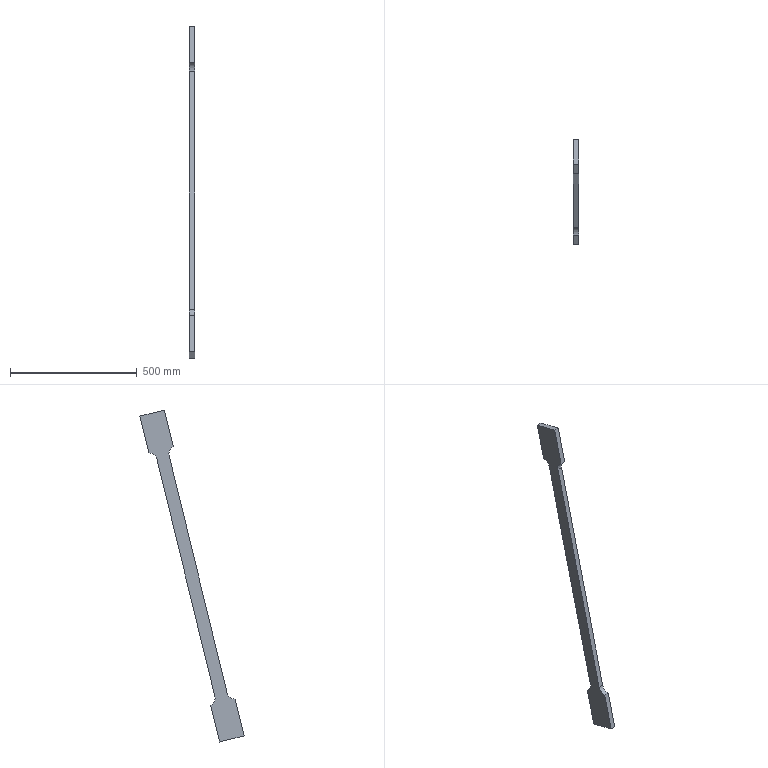Component | SolidWorks | Bocna spona oslonca izbacivaca-1 | 1 solid | 14 faces | box 20 x 412.18 x 1310.78 mm | volume 1639556 mm3 | plane 10 | cylinder 4 | commonest cylinder face diameters 60 x4
build123d program:
from build123d import *

# Parameters (mm, degrees)
BOSS_EXTRUDE1_DEPTH = 20


with BuildPart() as part:
    # Sketch1 → Boss-Extrude1 (new body)
    with BuildSketch(Plane(origin=(-5.82, 0, 0), x_dir=(0, 0, -1), z_dir=(1, 0, 0))):
        with BuildLine():
            Line((-662.5, 50), (-662.5, -50))
            Line((-662.5, -50), (-512.5, -50))
            ThreePointArc((-512.5, -50), (-502.285, -32.087), (-482.92, -25))
            Line((-482.92, -25), (482.92, -25))
            ThreePointArc((482.92, -25), (502.285, -32.087), (512.5, -50))
            Line((512.5, -50), (662.5, -50))
            Line((662.5, -50), (662.5, 50))
            Line((662.5, 50), (512.5, 50))
            ThreePointArc((512.5, 50), (502.285, 32.087), (482.92, 25))
            Line((482.92, 25), (-482.92, 25))
            ThreePointArc((-482.92, 25), (-502.285, 32.087), (-512.5, 50))
            Line((-512.5, 50), (-662.5, 50))
        make_face()
    extrude(amount=BOSS_EXTRUDE1_DEPTH)


solid = part.part

# Placed as in the assembly
solid = solid.moved(Location((6.82, 160.049, -734.493), (166.245, 0, 0)))
STEP:
#1=COLOUR_RGB('',0.7922,0.8196,0.9333);
#2=FILL_AREA_STYLE_COLOUR('',#1);
#3=FILL_AREA_STYLE('',(#2));
#4=SURFACE_STYLE_FILL_AREA(#3);
#5=SURFACE_SIDE_STYLE('',(#4));
#6=SURFACE_STYLE_USAGE(.BOTH.,#5);
#7=PRESENTATION_STYLE_ASSIGNMENT((#6));
#8=CARTESIAN_POINT('',(0.03937,3.416,-48.984));
#9=VERTEX_POINT('',#8);
#10=CARTESIAN_POINT('',(0.03937,2.737,-47.618));
#11=VERTEX_POINT('',#10);
#12=CARTESIAN_POINT('',(0.03937,3.884,-47.899));
#13=DIRECTION('',(-1.,-0.,-0.));
#14=DIRECTION('',(0.,-0.2378,-0.9713));
#15=AXIS2_PLACEMENT_3D('',#12,#13,#14);
#16=CIRCLE('',#15,1.181);
#17=EDGE_CURVE('',#9,#11,#16,.T.);
#18=ORIENTED_EDGE('',*,*,#17,.T.);
#19=CARTESIAN_POINT('',(0.8268,2.737,-47.618));
#20=VERTEX_POINT('',#19);
#21=CARTESIAN_POINT('',(0.8268,2.737,-47.618));
#22=DIRECTION('',(-1.,-0.,-0.));
#23=VECTOR('',#22,39.37);
#24=LINE('',#21,#23);
#25=EDGE_CURVE('',#20,#11,#24,.T.);
#26=ORIENTED_EDGE('',*,*,#25,.F.);
#27=CARTESIAN_POINT('',(0.8268,3.416,-48.984));
#28=VERTEX_POINT('',#27);
#29=CARTESIAN_POINT('',(0.8268,3.884,-47.899));
#30=DIRECTION('',(-1.,-0.,-0.));
#31=DIRECTION('',(0.,-0.2378,-0.9713));
#32=AXIS2_PLACEMENT_3D('',#29,#30,#31);
#33=CIRCLE('',#32,1.181);
#34=EDGE_CURVE('',#28,#20,#33,.T.);
#35=ORIENTED_EDGE('',*,*,#34,.F.);
#36=CARTESIAN_POINT('',(0.8268,3.416,-48.984));
#37=DIRECTION('',(-1.,-0.,-0.));
#38=VECTOR('',#37,39.37);
#39=LINE('',#36,#38);
#40=EDGE_CURVE('',#28,#9,#39,.T.);
#41=ORIENTED_EDGE('',*,*,#40,.T.);
#42=EDGE_LOOP('',(#18,#26,#35,#41));
#43=FACE_OUTER_BOUND('',#42,.T.);
#44=CARTESIAN_POINT('',(0.8268,3.884,-47.899));
#45=DIRECTION('',(-1.,-0.,-0.));
#46=DIRECTION('',(0.,0.2378,0.9713));
#47=AXIS2_PLACEMENT_3D('',#44,#45,#46);
#48=CYLINDRICAL_SURFACE('',#47,1.181);
#49=ADVANCED_FACE('',(#43),#48,.F.);
#50=CARTESIAN_POINT('',(0.03937,11.778,-10.684));
#51=VERTEX_POINT('',#50);
#52=CARTESIAN_POINT('',(0.03937,11.778,-10.684));
#53=DIRECTION('',(-0.,0.2378,0.9713));
#54=VECTOR('',#53,39.37);
#55=LINE('',#52,#54);
#56=EDGE_CURVE('',#11,#51,#55,.T.);
#57=ORIENTED_EDGE('',*,*,#56,.T.);
#58=CARTESIAN_POINT('',(0.8268,11.778,-10.684));
#59=VERTEX_POINT('',#58);
#60=CARTESIAN_POINT('',(0.8268,11.778,-10.684));
#61=DIRECTION('',(-1.,-0.,-0.));
#62=VECTOR('',#61,39.37);
#63=LINE('',#60,#62);
#64=EDGE_CURVE('',#59,#51,#63,.T.);
#65=ORIENTED_EDGE('',*,*,#64,.F.);
#66=CARTESIAN_POINT('',(0.8268,11.778,-10.684));
#67=DIRECTION('',(-0.,0.2378,0.9713));
#68=VECTOR('',#67,39.37);
#69=LINE('',#66,#68);
#70=EDGE_CURVE('',#20,#59,#69,.T.);
#71=ORIENTED_EDGE('',*,*,#70,.F.);
#72=ORIENTED_EDGE('',*,*,#25,.T.);
#73=EDGE_LOOP('',(#57,#65,#71,#72));
#74=FACE_OUTER_BOUND('',#73,.T.);
#75=CARTESIAN_POINT('',(0.8268,11.778,-10.684));
#76=DIRECTION('',(-0.,-0.9713,0.2378));
#77=DIRECTION('',(1.,-0.,0.));
#78=AXIS2_PLACEMENT_3D('',#75,#76,#77);
#79=PLANE('',#78);
#80=ADVANCED_FACE('',(#74),#79,.F.);
#81=CARTESIAN_POINT('',(0.03937,13.011,-9.787));
#82=VERTEX_POINT('',#81);
#83=CARTESIAN_POINT('',(0.03937,12.925,-10.965));
#84=DIRECTION('',(-1.,-0.,-0.));
#85=DIRECTION('',(-0.,0.2378,0.9713));
#86=AXIS2_PLACEMENT_3D('',#83,#84,#85);
#87=CIRCLE('',#86,1.181);
#88=EDGE_CURVE('',#51,#82,#87,.T.);
#89=ORIENTED_EDGE('',*,*,#88,.T.);
#90=CARTESIAN_POINT('',(0.8268,13.011,-9.787));
#91=VERTEX_POINT('',#90);
#92=CARTESIAN_POINT('',(0.8268,13.011,-9.787));
#93=DIRECTION('',(-1.,-0.,-0.));
#94=VECTOR('',#93,39.37);
#95=LINE('',#92,#94);
#96=EDGE_CURVE('',#91,#82,#95,.T.);
#97=ORIENTED_EDGE('',*,*,#96,.F.);
#98=CARTESIAN_POINT('',(0.8268,12.925,-10.965));
#99=DIRECTION('',(-1.,-0.,-0.));
#100=DIRECTION('',(0.,0.2378,0.9713));
#101=AXIS2_PLACEMENT_3D('',#98,#99,#100);
#102=CIRCLE('',#101,1.181);
#103=EDGE_CURVE('',#59,#91,#102,.T.);
#104=ORIENTED_EDGE('',*,*,#103,.F.);
#105=ORIENTED_EDGE('',*,*,#64,.T.);
#106=EDGE_LOOP('',(#89,#97,#104,#105));
#107=FACE_OUTER_BOUND('',#106,.T.);
#108=CARTESIAN_POINT('',(0.8268,12.925,-10.965));
#109=DIRECTION('',(-1.,-0.,-0.));
#110=DIRECTION('',(0.,0.2378,0.9713));
#111=AXIS2_PLACEMENT_3D('',#108,#109,#110);
#112=CYLINDRICAL_SURFACE('',#111,1.181);
#113=ADVANCED_FACE('',(#107),#112,.F.);
#114=CARTESIAN_POINT('',(0.03937,14.415,-4.05));
#115=VERTEX_POINT('',#114);
#116=CARTESIAN_POINT('',(0.03937,13.011,-9.787));
#117=DIRECTION('',(-0.,0.2378,0.9713));
#118=VECTOR('',#117,39.37);
#119=LINE('',#116,#118);
#120=EDGE_CURVE('',#82,#115,#119,.T.);
#121=ORIENTED_EDGE('',*,*,#120,.T.);
#122=CARTESIAN_POINT('',(0.8268,14.415,-4.05));
#123=VERTEX_POINT('',#122);
#124=CARTESIAN_POINT('',(0.8268,14.415,-4.05));
#125=DIRECTION('',(-1.,-0.,-0.));
#126=VECTOR('',#125,39.37);
#127=LINE('',#124,#126);
#128=EDGE_CURVE('',#123,#115,#127,.T.);
#129=ORIENTED_EDGE('',*,*,#128,.F.);
#130=CARTESIAN_POINT('',(0.8268,13.011,-9.787));
#131=DIRECTION('',(-0.,0.2378,0.9713));
#132=VECTOR('',#131,39.37);
#133=LINE('',#130,#132);
#134=EDGE_CURVE('',#91,#123,#133,.T.);
#135=ORIENTED_EDGE('',*,*,#134,.F.);
#136=ORIENTED_EDGE('',*,*,#96,.T.);
#137=EDGE_LOOP('',(#121,#129,#135,#136));
#138=FACE_OUTER_BOUND('',#137,.T.);
#139=CARTESIAN_POINT('',(0.8268,13.011,-9.787));
#140=DIRECTION('',(-0.,-0.9713,0.2378));
#141=DIRECTION('',(1.,-0.,0.));
#142=AXIS2_PLACEMENT_3D('',#139,#140,#141);
#143=PLANE('',#142);
#144=ADVANCED_FACE('',(#138),#143,.F.);
#145=CARTESIAN_POINT('',(0.03937,10.591,-3.114));
#146=VERTEX_POINT('',#145);
#147=CARTESIAN_POINT('',(0.03937,14.415,-4.05));
#148=DIRECTION('',(0.,-0.9713,0.2378));
#149=VECTOR('',#148,39.37);
#150=LINE('',#147,#149);
#151=EDGE_CURVE('',#115,#146,#150,.T.);
#152=ORIENTED_EDGE('',*,*,#151,.T.);
#153=CARTESIAN_POINT('',(0.8268,10.591,-3.114));
#154=VERTEX_POINT('',#153);
#155=CARTESIAN_POINT('',(0.8268,10.591,-3.114));
#156=DIRECTION('',(-1.,-0.,-0.));
#157=VECTOR('',#156,39.37);
#158=LINE('',#155,#157);
#159=EDGE_CURVE('',#154,#146,#158,.T.);
#160=ORIENTED_EDGE('',*,*,#159,.F.);
#161=CARTESIAN_POINT('',(0.8268,14.415,-4.05));
#162=DIRECTION('',(0.,-0.9713,0.2378));
#163=VECTOR('',#162,39.37);
#164=LINE('',#161,#163);
#165=EDGE_CURVE('',#123,#154,#164,.T.);
#166=ORIENTED_EDGE('',*,*,#165,.F.);
#167=ORIENTED_EDGE('',*,*,#128,.T.);
#168=EDGE_LOOP('',(#152,#160,#166,#167));
#169=FACE_OUTER_BOUND('',#168,.T.);
#170=CARTESIAN_POINT('',(0.8268,14.415,-4.05));
#171=DIRECTION('',(0.,-0.2378,-0.9713));
#172=DIRECTION('',(-1.,0.,-0.));
#173=AXIS2_PLACEMENT_3D('',#170,#171,#172);
#174=PLANE('',#173);
#175=ADVANCED_FACE('',(#169),#174,.F.);
#176=CARTESIAN_POINT('',(0.03937,9.187,-8.85));
#177=VERTEX_POINT('',#176);
#178=CARTESIAN_POINT('',(0.03937,9.187,-8.85));
#179=DIRECTION('',(0.,-0.2378,-0.9713));
#180=VECTOR('',#179,39.37);
#181=LINE('',#178,#180);
#182=EDGE_CURVE('',#146,#177,#181,.T.);
#183=ORIENTED_EDGE('',*,*,#182,.T.);
#184=CARTESIAN_POINT('',(0.8268,9.187,-8.85));
#185=VERTEX_POINT('',#184);
#186=CARTESIAN_POINT('',(0.8268,9.187,-8.85));
#187=DIRECTION('',(-1.,-0.,-0.));
#188=VECTOR('',#187,39.37);
#189=LINE('',#186,#188);
#190=EDGE_CURVE('',#185,#177,#189,.T.);
#191=ORIENTED_EDGE('',*,*,#190,.F.);
#192=CARTESIAN_POINT('',(0.8268,9.187,-8.85));
#193=DIRECTION('',(0.,-0.2378,-0.9713));
#194=VECTOR('',#193,39.37);
#195=LINE('',#192,#194);
#196=EDGE_CURVE('',#154,#185,#195,.T.);
#197=ORIENTED_EDGE('',*,*,#196,.F.);
#198=ORIENTED_EDGE('',*,*,#159,.T.);
#199=EDGE_LOOP('',(#183,#191,#197,#198));
#200=FACE_OUTER_BOUND('',#199,.T.);
#201=CARTESIAN_POINT('',(0.8268,9.187,-8.85));
#202=DIRECTION('',(0.,0.9713,-0.2378));
#203=DIRECTION('',(-0.,0.2378,0.9713));
#204=AXIS2_PLACEMENT_3D('',#201,#202,#203);
#205=PLANE('',#204);
#206=ADVANCED_FACE('',(#200),#205,.F.);
#207=CARTESIAN_POINT('',(0.03937,9.866,-10.216));
#208=VERTEX_POINT('',#207);
#209=CARTESIAN_POINT('',(0.03937,8.719,-9.935));
#210=DIRECTION('',(-1.,-0.,-0.));
#211=DIRECTION('',(0.,-0.2378,-0.9713));
#212=AXIS2_PLACEMENT_3D('',#209,#210,#211);
#213=CIRCLE('',#212,1.181);
#214=EDGE_CURVE('',#177,#208,#213,.T.);
#215=ORIENTED_EDGE('',*,*,#214,.T.);
#216=CARTESIAN_POINT('',(0.8268,9.866,-10.216));
#217=VERTEX_POINT('',#216);
#218=CARTESIAN_POINT('',(0.8268,9.866,-10.216));
#219=DIRECTION('',(-1.,-0.,-0.));
#220=VECTOR('',#219,39.37);
#221=LINE('',#218,#220);
#222=EDGE_CURVE('',#217,#208,#221,.T.);
#223=ORIENTED_EDGE('',*,*,#222,.F.);
#224=CARTESIAN_POINT('',(0.8268,8.719,-9.935));
#225=DIRECTION('',(-1.,-0.,-0.));
#226=DIRECTION('',(0.,-0.2378,-0.9713));
#227=AXIS2_PLACEMENT_3D('',#224,#225,#226);
#228=CIRCLE('',#227,1.181);
#229=EDGE_CURVE('',#185,#217,#228,.T.);
#230=ORIENTED_EDGE('',*,*,#229,.F.);
#231=ORIENTED_EDGE('',*,*,#190,.T.);
#232=EDGE_LOOP('',(#215,#223,#230,#231));
#233=FACE_OUTER_BOUND('',#232,.T.);
#234=CARTESIAN_POINT('',(0.8268,8.719,-9.935));
#235=DIRECTION('',(-1.,-0.,-0.));
#236=DIRECTION('',(0.,0.2378,0.9713));
#237=AXIS2_PLACEMENT_3D('',#234,#235,#236);
#238=CYLINDRICAL_SURFACE('',#237,1.181);
#239=ADVANCED_FACE('',(#233),#238,.F.);
#240=CARTESIAN_POINT('',(0.03937,0.8245,-47.15));
#241=VERTEX_POINT('',#240);
#242=CARTESIAN_POINT('',(0.03937,9.866,-10.216));
#243=DIRECTION('',(0.,-0.2378,-0.9713));
#244=VECTOR('',#243,39.37);
#245=LINE('',#242,#244);
#246=EDGE_CURVE('',#208,#241,#245,.T.);
#247=ORIENTED_EDGE('',*,*,#246,.T.);
#248=CARTESIAN_POINT('',(0.8268,0.8245,-47.15));
#249=VERTEX_POINT('',#248);
#250=CARTESIAN_POINT('',(0.8268,0.8245,-47.15));
#251=DIRECTION('',(-1.,-0.,-0.));
#252=VECTOR('',#251,39.37);
#253=LINE('',#250,#252);
#254=EDGE_CURVE('',#249,#241,#253,.T.);
#255=ORIENTED_EDGE('',*,*,#254,.F.);
#256=CARTESIAN_POINT('',(0.8268,9.866,-10.216));
#257=DIRECTION('',(0.,-0.2378,-0.9713));
#258=VECTOR('',#257,39.37);
#259=LINE('',#256,#258);
#260=EDGE_CURVE('',#217,#249,#259,.T.);
#261=ORIENTED_EDGE('',*,*,#260,.F.);
#262=ORIENTED_EDGE('',*,*,#222,.T.);
#263=EDGE_LOOP('',(#247,#255,#261,#262));
#264=FACE_OUTER_BOUND('',#263,.T.);
#265=CARTESIAN_POINT('',(0.8268,9.866,-10.216));
#266=DIRECTION('',(0.,0.9713,-0.2378));
#267=DIRECTION('',(-1.,0.,-0.));
#268=AXIS2_PLACEMENT_3D('',#265,#266,#267);
#269=PLANE('',#268);
#270=ADVANCED_FACE('',(#264),#269,.F.);
#271=CARTESIAN_POINT('',(0.03937,-0.4084,-48.048));
#272=VERTEX_POINT('',#271);
#273=CARTESIAN_POINT('',(0.03937,-0.3227,-46.87));
#274=DIRECTION('',(-1.,-0.,-0.));
#275=DIRECTION('',(-0.,0.2378,0.9713));
#276=AXIS2_PLACEMENT_3D('',#273,#274,#275);
#277=CIRCLE('',#276,1.181);
#278=EDGE_CURVE('',#241,#272,#277,.T.);
#279=ORIENTED_EDGE('',*,*,#278,.T.);
#280=CARTESIAN_POINT('',(0.8268,-0.4084,-48.048));
#281=VERTEX_POINT('',#280);
#282=CARTESIAN_POINT('',(0.8268,-0.4084,-48.048));
#283=DIRECTION('',(-1.,-0.,-0.));
#284=VECTOR('',#283,39.37);
#285=LINE('',#282,#284);
#286=EDGE_CURVE('',#281,#272,#285,.T.);
#287=ORIENTED_EDGE('',*,*,#286,.F.);
#288=CARTESIAN_POINT('',(0.8268,-0.3227,-46.87));
#289=DIRECTION('',(-1.,-0.,-0.));
#290=DIRECTION('',(0.,0.2378,0.9713));
#291=AXIS2_PLACEMENT_3D('',#288,#289,#290);
#292=CIRCLE('',#291,1.181);
#293=EDGE_CURVE('',#249,#281,#292,.T.);
#294=ORIENTED_EDGE('',*,*,#293,.F.);
#295=ORIENTED_EDGE('',*,*,#254,.T.);
#296=EDGE_LOOP('',(#279,#287,#294,#295));
#297=FACE_OUTER_BOUND('',#296,.T.);
#298=CARTESIAN_POINT('',(0.8268,-0.3227,-46.87));
#299=DIRECTION('',(-1.,-0.,-0.));
#300=DIRECTION('',(0.,0.2378,0.9713));
#301=AXIS2_PLACEMENT_3D('',#298,#299,#300);
#302=CYLINDRICAL_SURFACE('',#301,1.181);
#303=ADVANCED_FACE('',(#297),#302,.F.);
#304=CARTESIAN_POINT('',(0.03937,-1.813,-53.784));
#305=VERTEX_POINT('',#304);
#306=CARTESIAN_POINT('',(0.03937,-0.4084,-48.048));
#307=DIRECTION('',(0.,-0.2378,-0.9713));
#308=VECTOR('',#307,39.37);
#309=LINE('',#306,#308);
#310=EDGE_CURVE('',#272,#305,#309,.T.);
#311=ORIENTED_EDGE('',*,*,#310,.T.);
#312=CARTESIAN_POINT('',(0.8268,-1.813,-53.784));
#313=VERTEX_POINT('',#312);
#314=CARTESIAN_POINT('',(0.8268,-1.813,-53.784));
#315=DIRECTION('',(-1.,-0.,-0.));
#316=VECTOR('',#315,39.37);
#317=LINE('',#314,#316);
#318=EDGE_CURVE('',#313,#305,#317,.T.);
#319=ORIENTED_EDGE('',*,*,#318,.F.);
#320=CARTESIAN_POINT('',(0.8268,-0.4084,-48.048));
#321=DIRECTION('',(0.,-0.2378,-0.9713));
#322=VECTOR('',#321,39.37);
#323=LINE('',#320,#322);
#324=EDGE_CURVE('',#281,#313,#323,.T.);
#325=ORIENTED_EDGE('',*,*,#324,.F.);
#326=ORIENTED_EDGE('',*,*,#286,.T.);
#327=EDGE_LOOP('',(#311,#319,#325,#326));
#328=FACE_OUTER_BOUND('',#327,.T.);
#329=CARTESIAN_POINT('',(0.8268,-0.4084,-48.048));
#330=DIRECTION('',(0.,0.9713,-0.2378));
#331=DIRECTION('',(-0.,0.2378,0.9713));
#332=AXIS2_PLACEMENT_3D('',#329,#330,#331);
#333=PLANE('',#332);
#334=ADVANCED_FACE('',(#328),#333,.F.);
#335=CARTESIAN_POINT('',(0.03937,2.012,-54.72));
#336=VERTEX_POINT('',#335);
#337=CARTESIAN_POINT('',(0.03937,2.012,-54.72));
#338=DIRECTION('',(-0.,0.9713,-0.2378));
#339=VECTOR('',#338,39.37);
#340=LINE('',#337,#339);
#341=EDGE_CURVE('',#305,#336,#340,.T.);
#342=ORIENTED_EDGE('',*,*,#341,.T.);
#343=CARTESIAN_POINT('',(0.8268,2.012,-54.72));
#344=VERTEX_POINT('',#343);
#345=CARTESIAN_POINT('',(0.8268,2.012,-54.72));
#346=DIRECTION('',(-1.,-0.,-0.));
#347=VECTOR('',#346,39.37);
#348=LINE('',#345,#347);
#349=EDGE_CURVE('',#344,#336,#348,.T.);
#350=ORIENTED_EDGE('',*,*,#349,.F.);
#351=CARTESIAN_POINT('',(0.8268,2.012,-54.72));
#352=DIRECTION('',(-0.,0.9713,-0.2378));
#353=VECTOR('',#352,39.37);
#354=LINE('',#351,#353);
#355=EDGE_CURVE('',#313,#344,#354,.T.);
#356=ORIENTED_EDGE('',*,*,#355,.F.);
#357=ORIENTED_EDGE('',*,*,#318,.T.);
#358=EDGE_LOOP('',(#342,#350,#356,#357));
#359=FACE_OUTER_BOUND('',#358,.T.);
#360=CARTESIAN_POINT('',(0.8268,2.012,-54.72));
#361=DIRECTION('',(-0.,0.2378,0.9713));
#362=DIRECTION('',(1.,-0.,0.));
#363=AXIS2_PLACEMENT_3D('',#360,#361,#362);
#364=PLANE('',#363);
#365=ADVANCED_FACE('',(#359),#364,.F.);
#366=CARTESIAN_POINT('',(0.03937,3.416,-48.984));
#367=DIRECTION('',(-0.,0.2378,0.9713));
#368=VECTOR('',#367,39.37);
#369=LINE('',#366,#368);
#370=EDGE_CURVE('',#336,#9,#369,.T.);
#371=ORIENTED_EDGE('',*,*,#370,.T.);
#372=ORIENTED_EDGE('',*,*,#40,.F.);
#373=CARTESIAN_POINT('',(0.8268,3.416,-48.984));
#374=DIRECTION('',(-0.,0.2378,0.9713));
#375=VECTOR('',#374,39.37);
#376=LINE('',#373,#375);
#377=EDGE_CURVE('',#344,#28,#376,.T.);
#378=ORIENTED_EDGE('',*,*,#377,.F.);
#379=ORIENTED_EDGE('',*,*,#349,.T.);
#380=EDGE_LOOP('',(#371,#372,#378,#379));
#381=FACE_OUTER_BOUND('',#380,.T.);
#382=CARTESIAN_POINT('',(0.8268,3.416,-48.984));
#383=DIRECTION('',(-0.,-0.9713,0.2378));
#384=DIRECTION('',(1.,-0.,0.));
#385=AXIS2_PLACEMENT_3D('',#382,#383,#384);
#386=PLANE('',#385);
#387=ADVANCED_FACE('',(#381),#386,.F.);
#388=ORIENTED_EDGE('',*,*,#34,.T.);
#389=ORIENTED_EDGE('',*,*,#70,.T.);
#390=ORIENTED_EDGE('',*,*,#103,.T.);
#391=ORIENTED_EDGE('',*,*,#134,.T.);
#392=ORIENTED_EDGE('',*,*,#165,.T.);
#393=ORIENTED_EDGE('',*,*,#196,.T.);
#394=ORIENTED_EDGE('',*,*,#229,.T.);
#395=ORIENTED_EDGE('',*,*,#260,.T.);
#396=ORIENTED_EDGE('',*,*,#293,.T.);
#397=ORIENTED_EDGE('',*,*,#324,.T.);
#398=ORIENTED_EDGE('',*,*,#355,.T.);
#399=ORIENTED_EDGE('',*,*,#377,.T.);
#400=EDGE_LOOP('',(#388,#389,#390,#391,#392,#393,#394,#395,#396,#397,#398,#399));
#401=FACE_OUTER_BOUND('',#400,.T.);
#402=CARTESIAN_POINT('',(0.8268,3.884,-47.899));
#403=DIRECTION('',(1.,0.,0.));
#404=DIRECTION('',(0.,-0.2378,-0.9713));
#405=AXIS2_PLACEMENT_3D('',#402,#403,#404);
#406=PLANE('',#405);
#407=ADVANCED_FACE('',(#401),#406,.T.);
#408=ORIENTED_EDGE('',*,*,#17,.F.);
#409=ORIENTED_EDGE('',*,*,#370,.F.);
#410=ORIENTED_EDGE('',*,*,#341,.F.);
#411=ORIENTED_EDGE('',*,*,#310,.F.);
#412=ORIENTED_EDGE('',*,*,#278,.F.);
#413=ORIENTED_EDGE('',*,*,#246,.F.);
#414=ORIENTED_EDGE('',*,*,#214,.F.);
#415=ORIENTED_EDGE('',*,*,#182,.F.);
#416=ORIENTED_EDGE('',*,*,#151,.F.);
#417=ORIENTED_EDGE('',*,*,#120,.F.);
#418=ORIENTED_EDGE('',*,*,#88,.F.);
#419=ORIENTED_EDGE('',*,*,#56,.F.);
#420=EDGE_LOOP('',(#408,#409,#410,#411,#412,#413,#414,#415,#416,#417,#418,#419));
#421=FACE_OUTER_BOUND('',#420,.T.);
#422=CARTESIAN_POINT('',(0.03937,3.884,-47.899));
#423=DIRECTION('',(1.,0.,0.));
#424=DIRECTION('',(0.,-0.2378,-0.9713));
#425=AXIS2_PLACEMENT_3D('',#422,#423,#424);
#426=PLANE('',#425);
#427=ADVANCED_FACE('',(#421),#426,.F.);
#428=CLOSED_SHELL('',(#49,#80,#113,#144,#175,#206,#239,#270,#303,#334,#365,#387,#407,#427));
#429=MANIFOLD_SOLID_BREP('',#428);
#430=STYLED_ITEM('',(#7),#429);
#431=PRESENTATION_LAYER_ASSIGNMENT('','',(#430));
#432=(LENGTH_UNIT()NAMED_UNIT(*)SI_UNIT($,.METRE.));
#433=LENGTH_MEASURE_WITH_UNIT(LENGTH_MEASURE(0.0254),#432);
#434=DIMENSIONAL_EXPONENTS(1.,0.,0.,0.,0.,0.,0.);
#435=(CONVERSION_BASED_UNIT('',#433)LENGTH_UNIT()NAMED_UNIT(#434));
#436=UNCERTAINTY_MEASURE_WITH_UNIT(LENGTH_MEASURE(0.00001),#435,'','');
#437=(NAMED_UNIT(*)PLANE_ANGLE_UNIT()SI_UNIT($,.RADIAN.));
#438=(NAMED_UNIT(*)SI_UNIT($,.STERADIAN.)SOLID_ANGLE_UNIT());
#439=(GEOMETRIC_REPRESENTATION_CONTEXT(3)GLOBAL_UNCERTAINTY_ASSIGNED_CONTEXT((#436))GLOBAL_UNIT_ASSIGNED_CONTEXT((#435,#437,#438))REPRESENTATION_CONTEXT('',''));
#440=MECHANICAL_DESIGN_GEOMETRIC_PRESENTATION_REPRESENTATION('',(#430),#439);
#441=CARTESIAN_POINT('',(0.,0.,0.));
#442=DIRECTION('',(0.,0.,1.));
#443=DIRECTION('',(1.,0.,0.));
#444=AXIS2_PLACEMENT_3D('',#441,#442,#443);
#445=(LENGTH_UNIT()NAMED_UNIT(*)SI_UNIT($,.METRE.));
#446=LENGTH_MEASURE_WITH_UNIT(LENGTH_MEASURE(0.0254),#445);
#447=DIMENSIONAL_EXPONENTS(1.,0.,0.,0.,0.,0.,0.);
#448=(CONVERSION_BASED_UNIT('',#446)LENGTH_UNIT()NAMED_UNIT(#447));
#449=UNCERTAINTY_MEASURE_WITH_UNIT(LENGTH_MEASURE(0.00001),#448,'','');
#450=(NAMED_UNIT(*)PLANE_ANGLE_UNIT()SI_UNIT($,.RADIAN.));
#451=(NAMED_UNIT(*)SI_UNIT($,.STERADIAN.)SOLID_ANGLE_UNIT());
#452=(GEOMETRIC_REPRESENTATION_CONTEXT(3)GLOBAL_UNCERTAINTY_ASSIGNED_CONTEXT((#449))GLOBAL_UNIT_ASSIGNED_CONTEXT((#448,#450,#451))REPRESENTATION_CONTEXT('',''));
#453=ADVANCED_BREP_SHAPE_REPRESENTATION('',(#429,#444),#452);